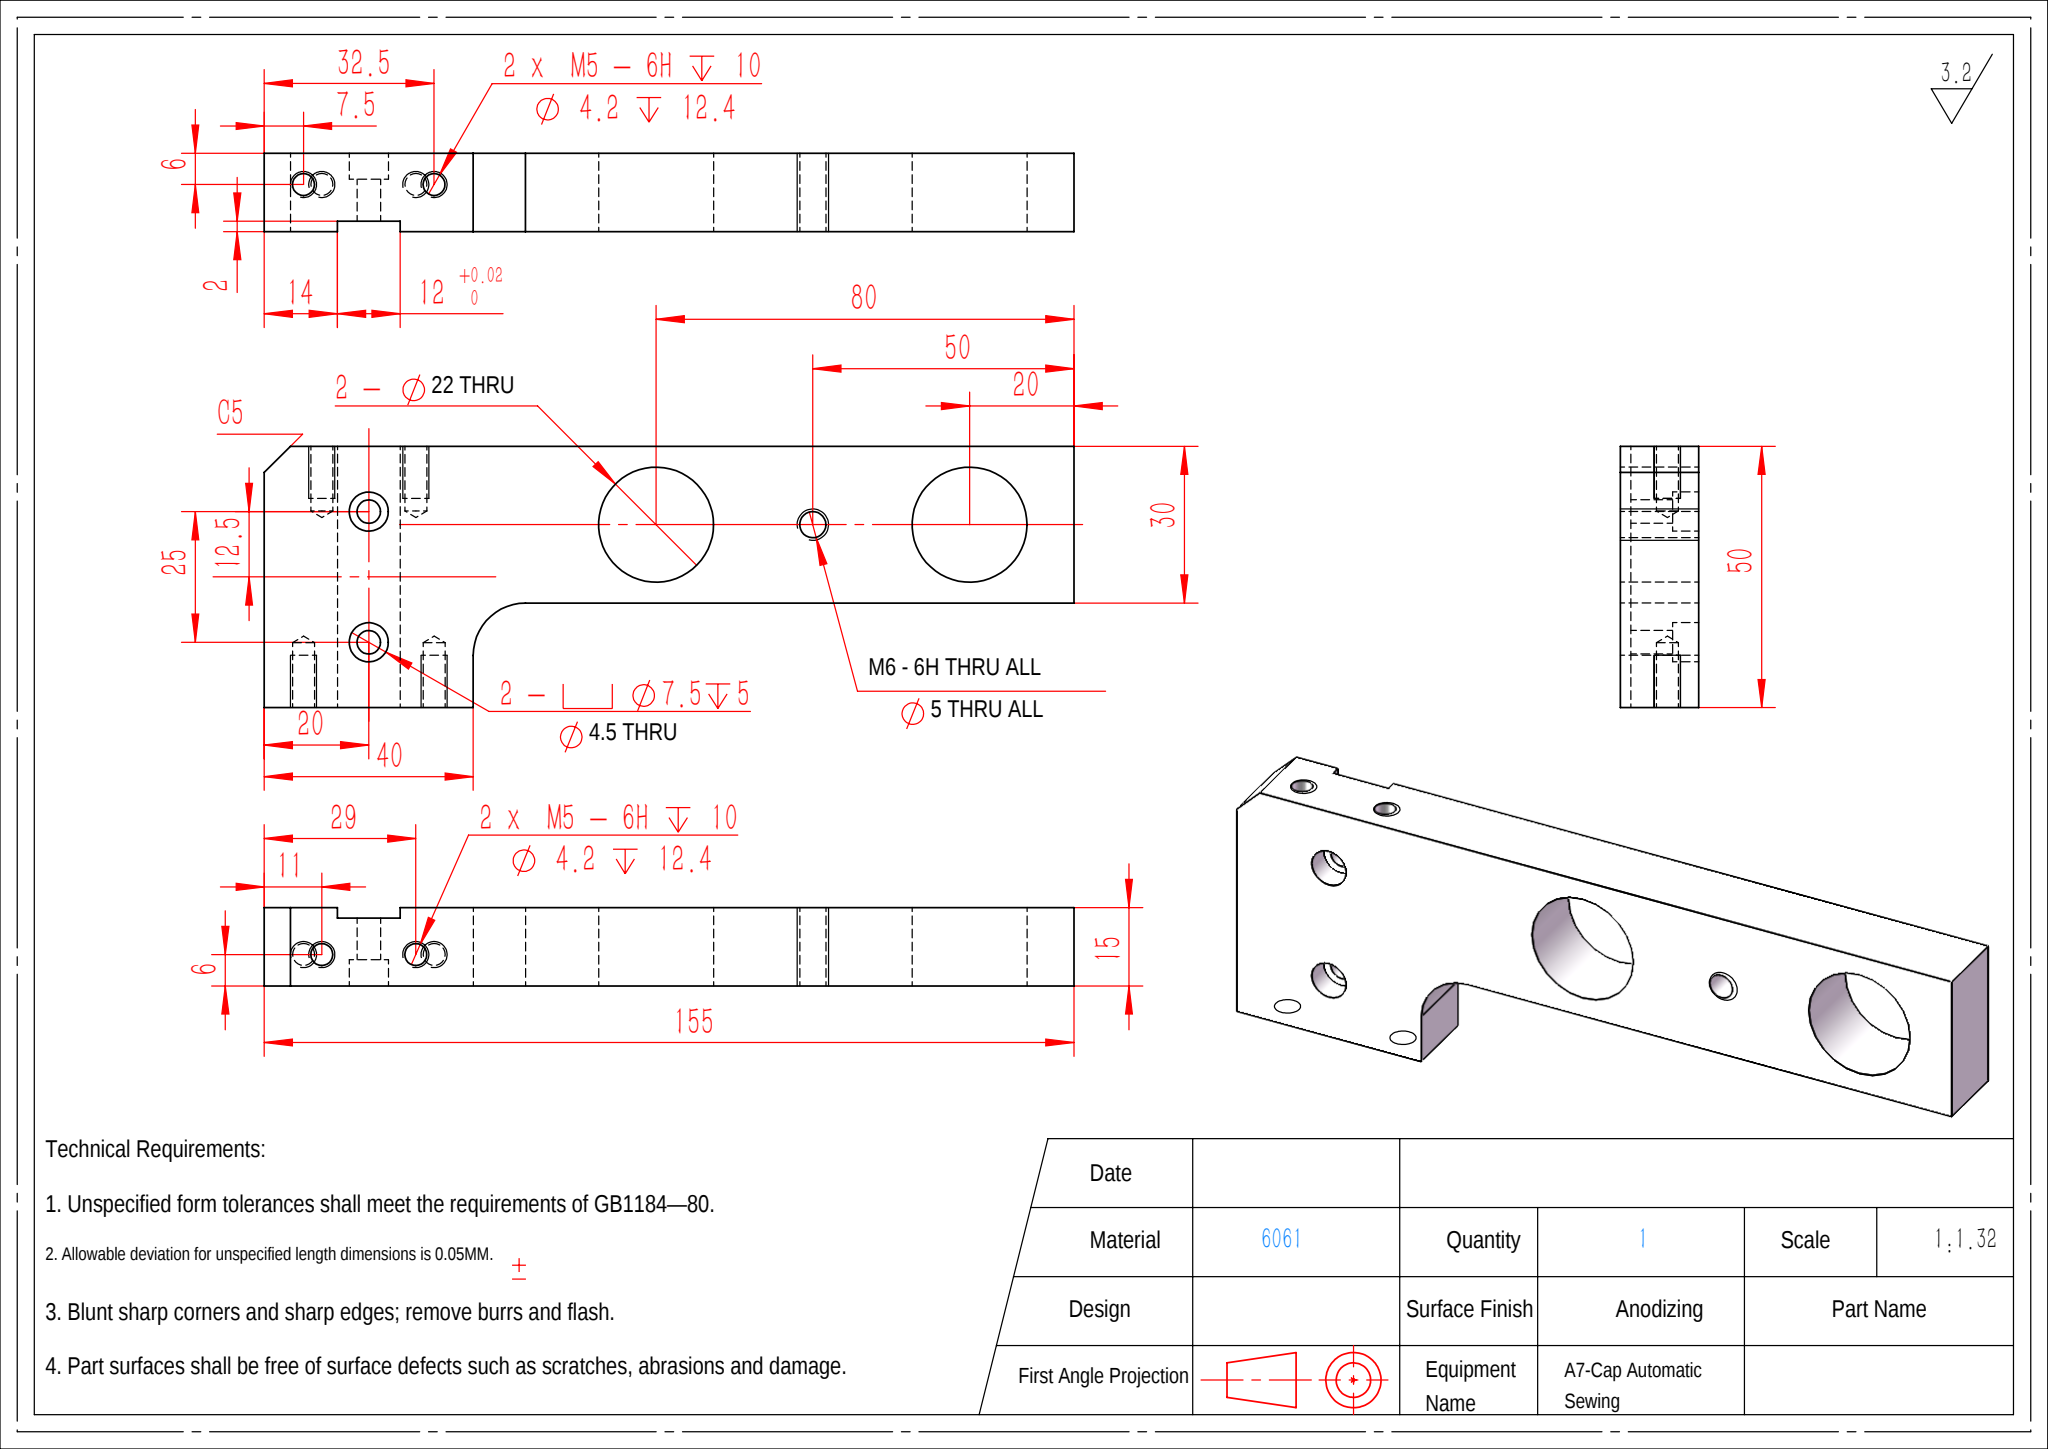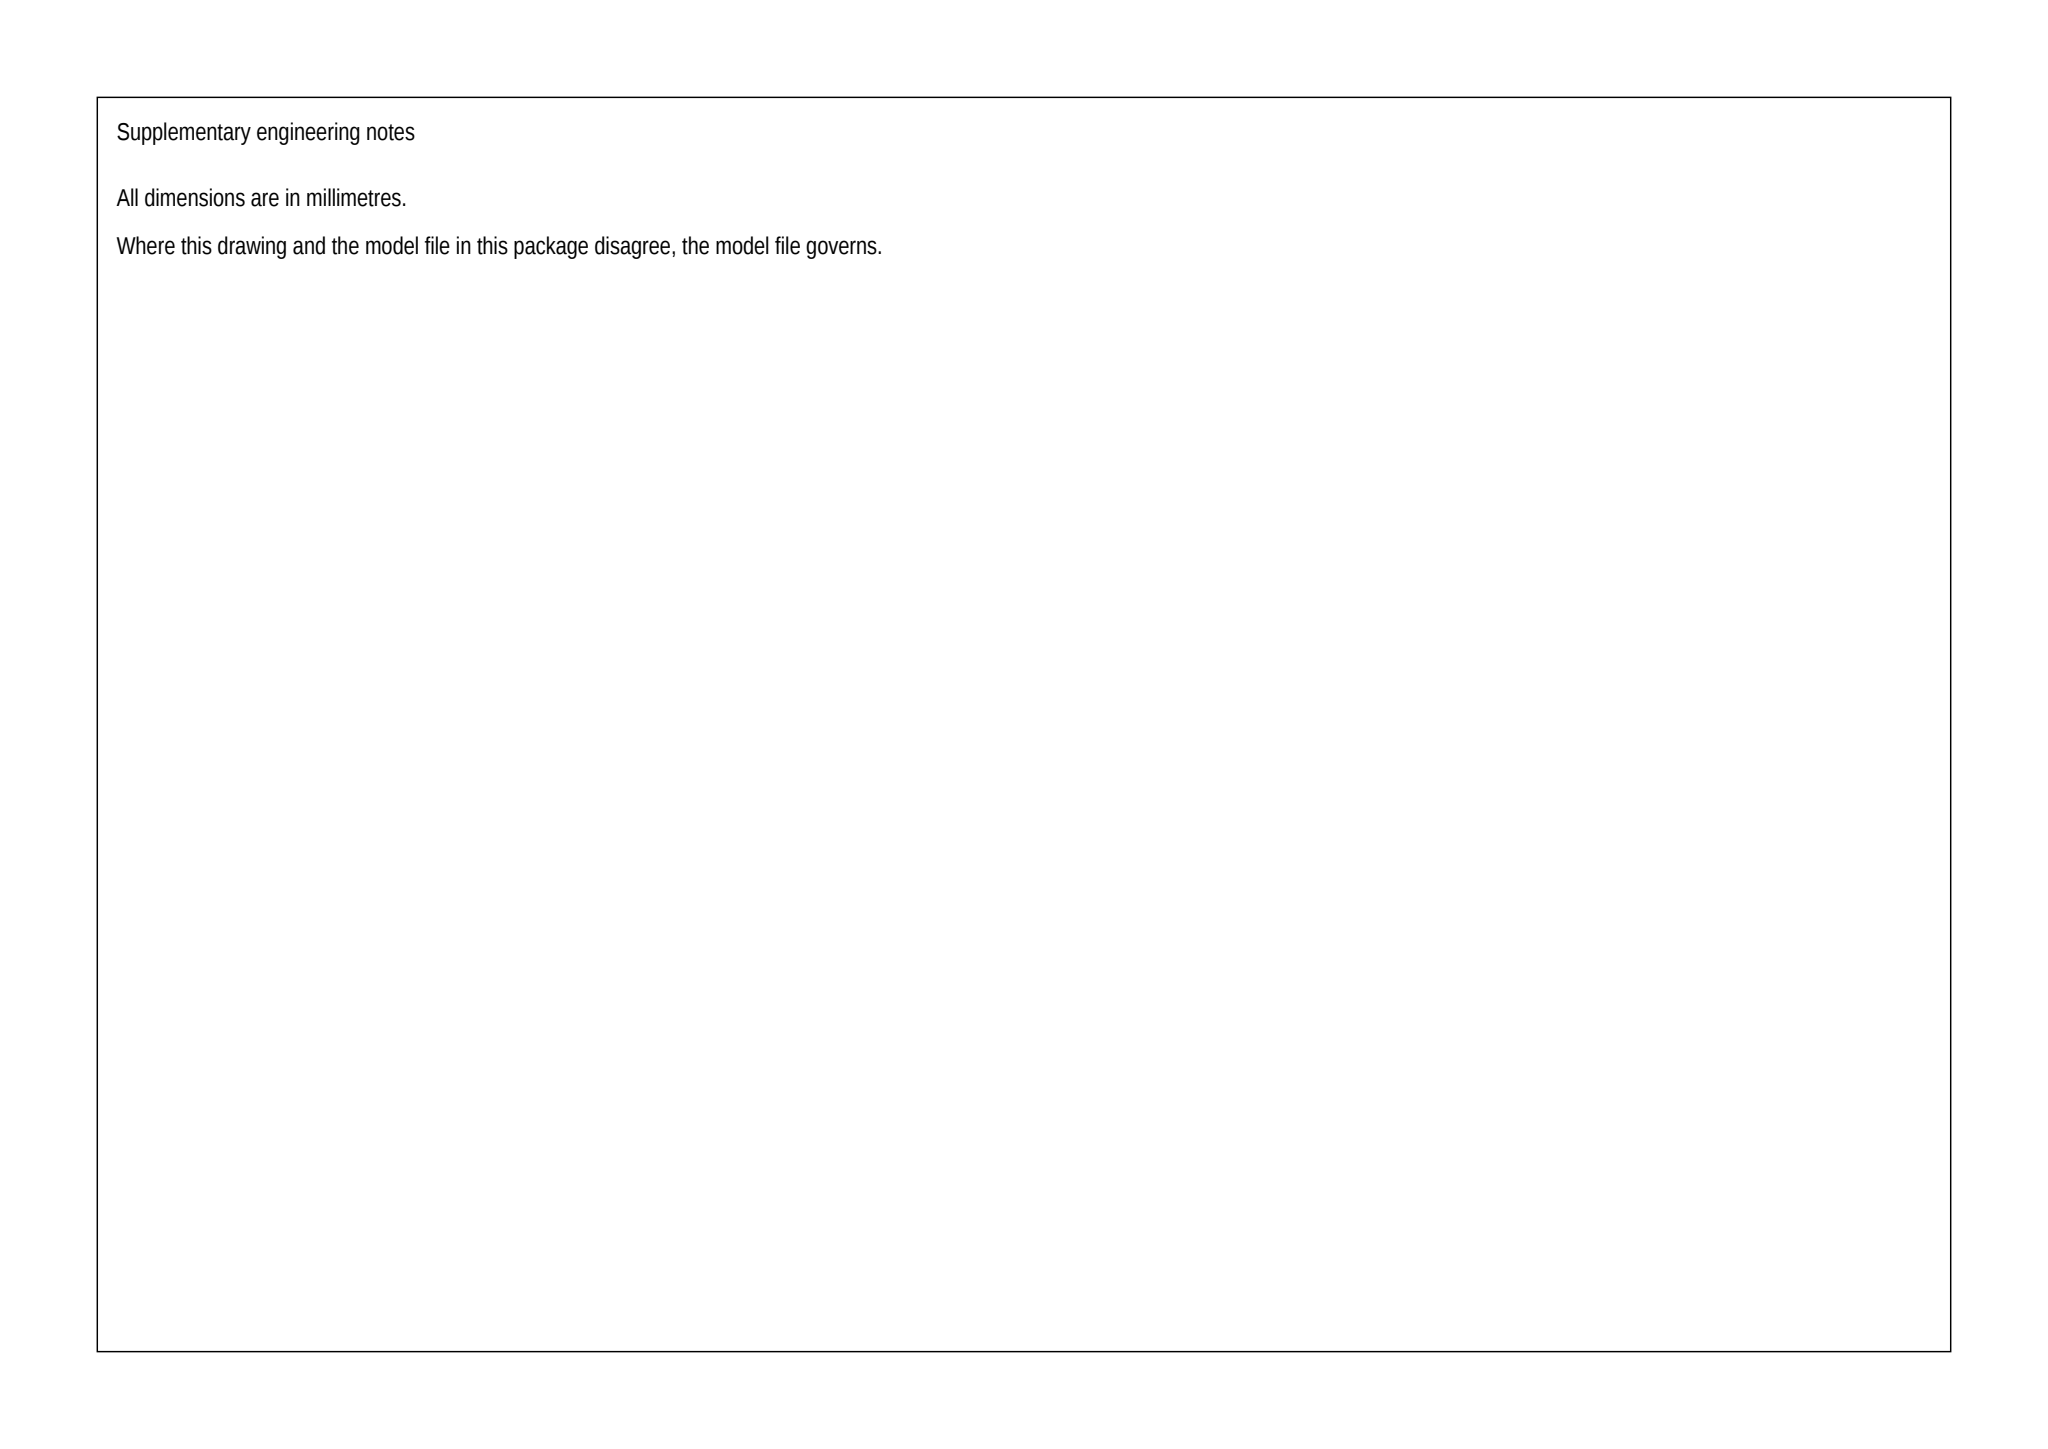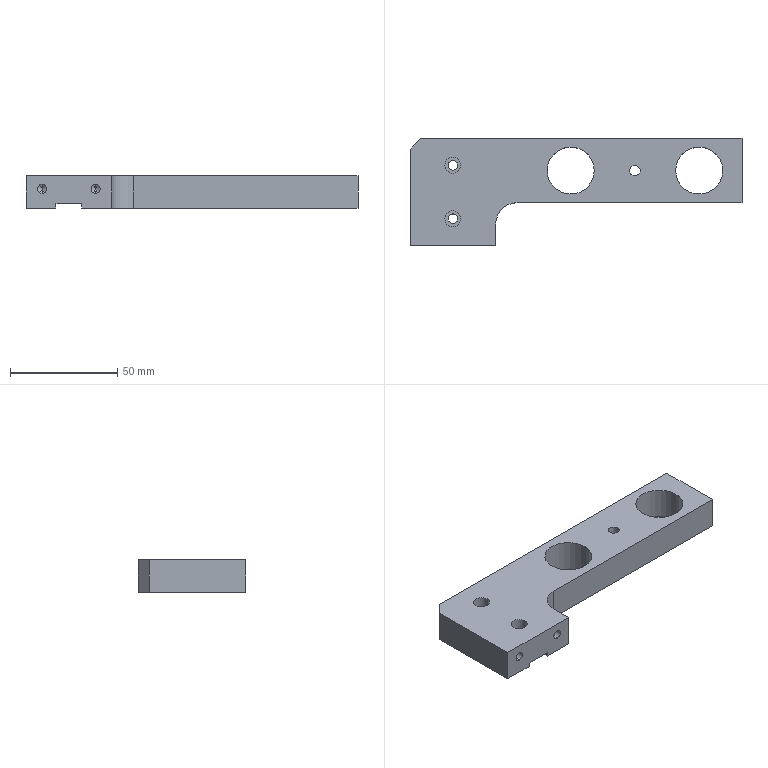Part | SolidWorks | mm | material 6061 | 1 solid | 46 faces | box 155 x 50 x 15 mm | volume 67579 mm3 | cylinder 23 | plane 15 | cone 8 | commonest cylinder face diameters 4.2 x8 7.5 x4 22 x4 4.5 x4 5 x2 20 x1
build123d program:
from build123d import *

# Parameters (mm, degrees)
SKETCH1_W             = 155
SKETCH1_H             = 15
BOSS_EXTRUDE1_DEPTH   = 15
SKETCH2_R             = 11
CUT_EXTRUDE1_DEPTH    = 81.351
SKETCH3_W             = 40
SKETCH3_H             = 15
BOSS_EXTRUDE2_DEPTH   = 20
SKETCH4_W             = 12
SKETCH4_H             = 50
CUT_EXTRUDE2_DEPTH    = 2
SKETCH5_R             = 2.25
CUT_EXTRUDE3_DEPTH    = 87.025
SKETCH6_R             = 3.75
CUT_EXTRUDE4_DEPTH    = 5
CHAMFER1_SIZE         = 5
M5_TAPPED_HOLE1_D     = 4.2
M5_TAPPED_HOLE1_DEPTH = 12.4
M5_TAPPED_HOLE1_TIP   = 1.262
M5_TAPPED_HOLE2_D     = 4.2
M5_TAPPED_HOLE2_DEPTH = 12.4
M5_TAPPED_HOLE2_TIP   = 1.262
FILLET1_R             = 10
M6_TAPPED_HOLE1_D     = 5


with BuildPart() as part:
    # Sketch1 → Boss-Extrude1 (new, symmetric)
    with BuildSketch(Plane(origin=(0, 0, 0), x_dir=(1, 0, 0), z_dir=(0, 1, 0))):
        Rectangle(SKETCH1_W, SKETCH1_H)
    extrude(amount=BOSS_EXTRUDE1_DEPTH, both=True)

    # Sketch2 → Cut-Extrude1 (cut, through all)
    with BuildSketch(Plane.XY.offset(7.5)):
        with Locations((57.5, 0)):
            Circle(SKETCH2_R)
        with Locations((-2.5, 0)):
            Circle(SKETCH2_R)
    extrude(amount=-CUT_EXTRUDE1_DEPTH, mode=Mode.SUBTRACT)

    # Sketch3 → Boss-Extrude2 (add)
    with BuildSketch(Plane(origin=(0, -15, 0), x_dir=(-1, 0, 0), z_dir=(0, -1, 0))):
        with Locations((57.5, 0)):
            Rectangle(SKETCH3_W, SKETCH3_H)
    extrude(amount=BOSS_EXTRUDE2_DEPTH)

    # Sketch4 → Cut-Extrude2 (cut)
    with BuildSketch(Plane(origin=(0, 0, -7.5), x_dir=(-1, 0, 0), z_dir=(0, 0, -1))):
        with Locations((57.5, -10)):
            Rectangle(SKETCH4_W, SKETCH4_H)
    extrude(amount=-CUT_EXTRUDE2_DEPTH, mode=Mode.SUBTRACT)

    # Sketch5 → Cut-Extrude3 (cut, through all)
    with BuildSketch(Plane(origin=(0, 0, -5.5), x_dir=(-1, 0, 0), z_dir=(0, 0, -1))):
        with Locations((57.5, 2.5)):
            Circle(SKETCH5_R)
        with Locations((57.5, -22.5)):
            Circle(SKETCH5_R)
    extrude(amount=-CUT_EXTRUDE3_DEPTH, mode=Mode.SUBTRACT)

    # Sketch6 → Cut-Extrude4 (cut)
    with BuildSketch(Plane.XY.offset(7.5)):
        with Locations((-57.5, 2.5)):
            Circle(SKETCH6_R)
        with Locations((-57.5, -22.5)):
            Circle(SKETCH6_R)
    extrude(amount=-CUT_EXTRUDE4_DEPTH, mode=Mode.SUBTRACT)

    # Chamfer1
    chamfer1_edges = [part.edges().sort_by_distance(p)[0] for p in [
        (-77.5, 15, 0),
    ]]
    chamfer(chamfer1_edges, length=CHAMFER1_SIZE)

    # M5 Tapped Hole1
    with Locations(Plane(origin=(-70, -35, 1.5), x_dir=(0, 0, -1), z_dir=(0, -1, 0))):
        with Locations((0, 0), (0, 25)):
            Hole(M5_TAPPED_HOLE1_D / 2, depth=M5_TAPPED_HOLE1_DEPTH)
            with Locations((0, 0, -(M5_TAPPED_HOLE1_DEPTH + M5_TAPPED_HOLE1_TIP / 2))):  # 118° drill point
                Cone(0, M5_TAPPED_HOLE1_D / 2, M5_TAPPED_HOLE1_TIP, mode=Mode.SUBTRACT)

    # M5 Tapped Hole2
    with Locations(Plane(origin=(-66.5, 15, 1.5), x_dir=(0, 0, 1), z_dir=(0, 1, 0))):
        with Locations((0, 0), (0, 18)):
            Hole(M5_TAPPED_HOLE2_D / 2, depth=M5_TAPPED_HOLE2_DEPTH)
            with Locations((0, 0, -(M5_TAPPED_HOLE2_DEPTH + M5_TAPPED_HOLE2_TIP / 2))):  # 118° drill point
                Cone(0, M5_TAPPED_HOLE2_D / 2, M5_TAPPED_HOLE2_TIP, mode=Mode.SUBTRACT)

    # Fillet1
    fillet1_edges = [part.edges().sort_by_distance(p)[0] for p in [
        (-37.5, -15, 0),
    ]]
    fillet(fillet1_edges, radius=FILLET1_R)

    # M6 Tapped Hole1 (through all)
    with Locations(Plane(origin=(27.5, 0, 7.5), x_dir=(1, 0, 0), z_dir=(0, 0, 1))):
        with Locations((0, 0)):
            Hole(M6_TAPPED_HOLE1_D / 2)


solid = part.part